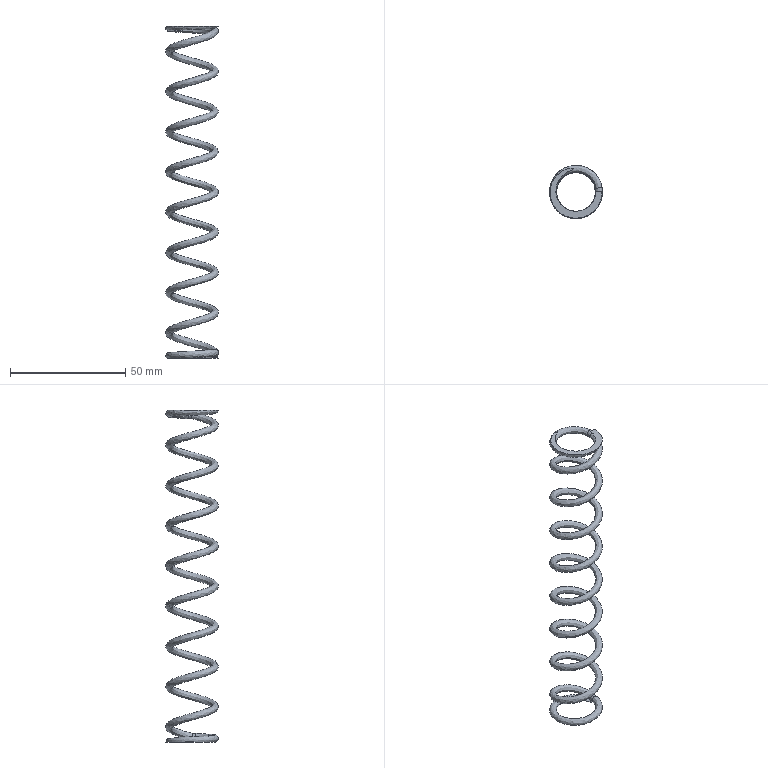Component | NX | SPRING | 1 solid | 9 faces | volume 4198 mm3 | spline 5 | plane 4